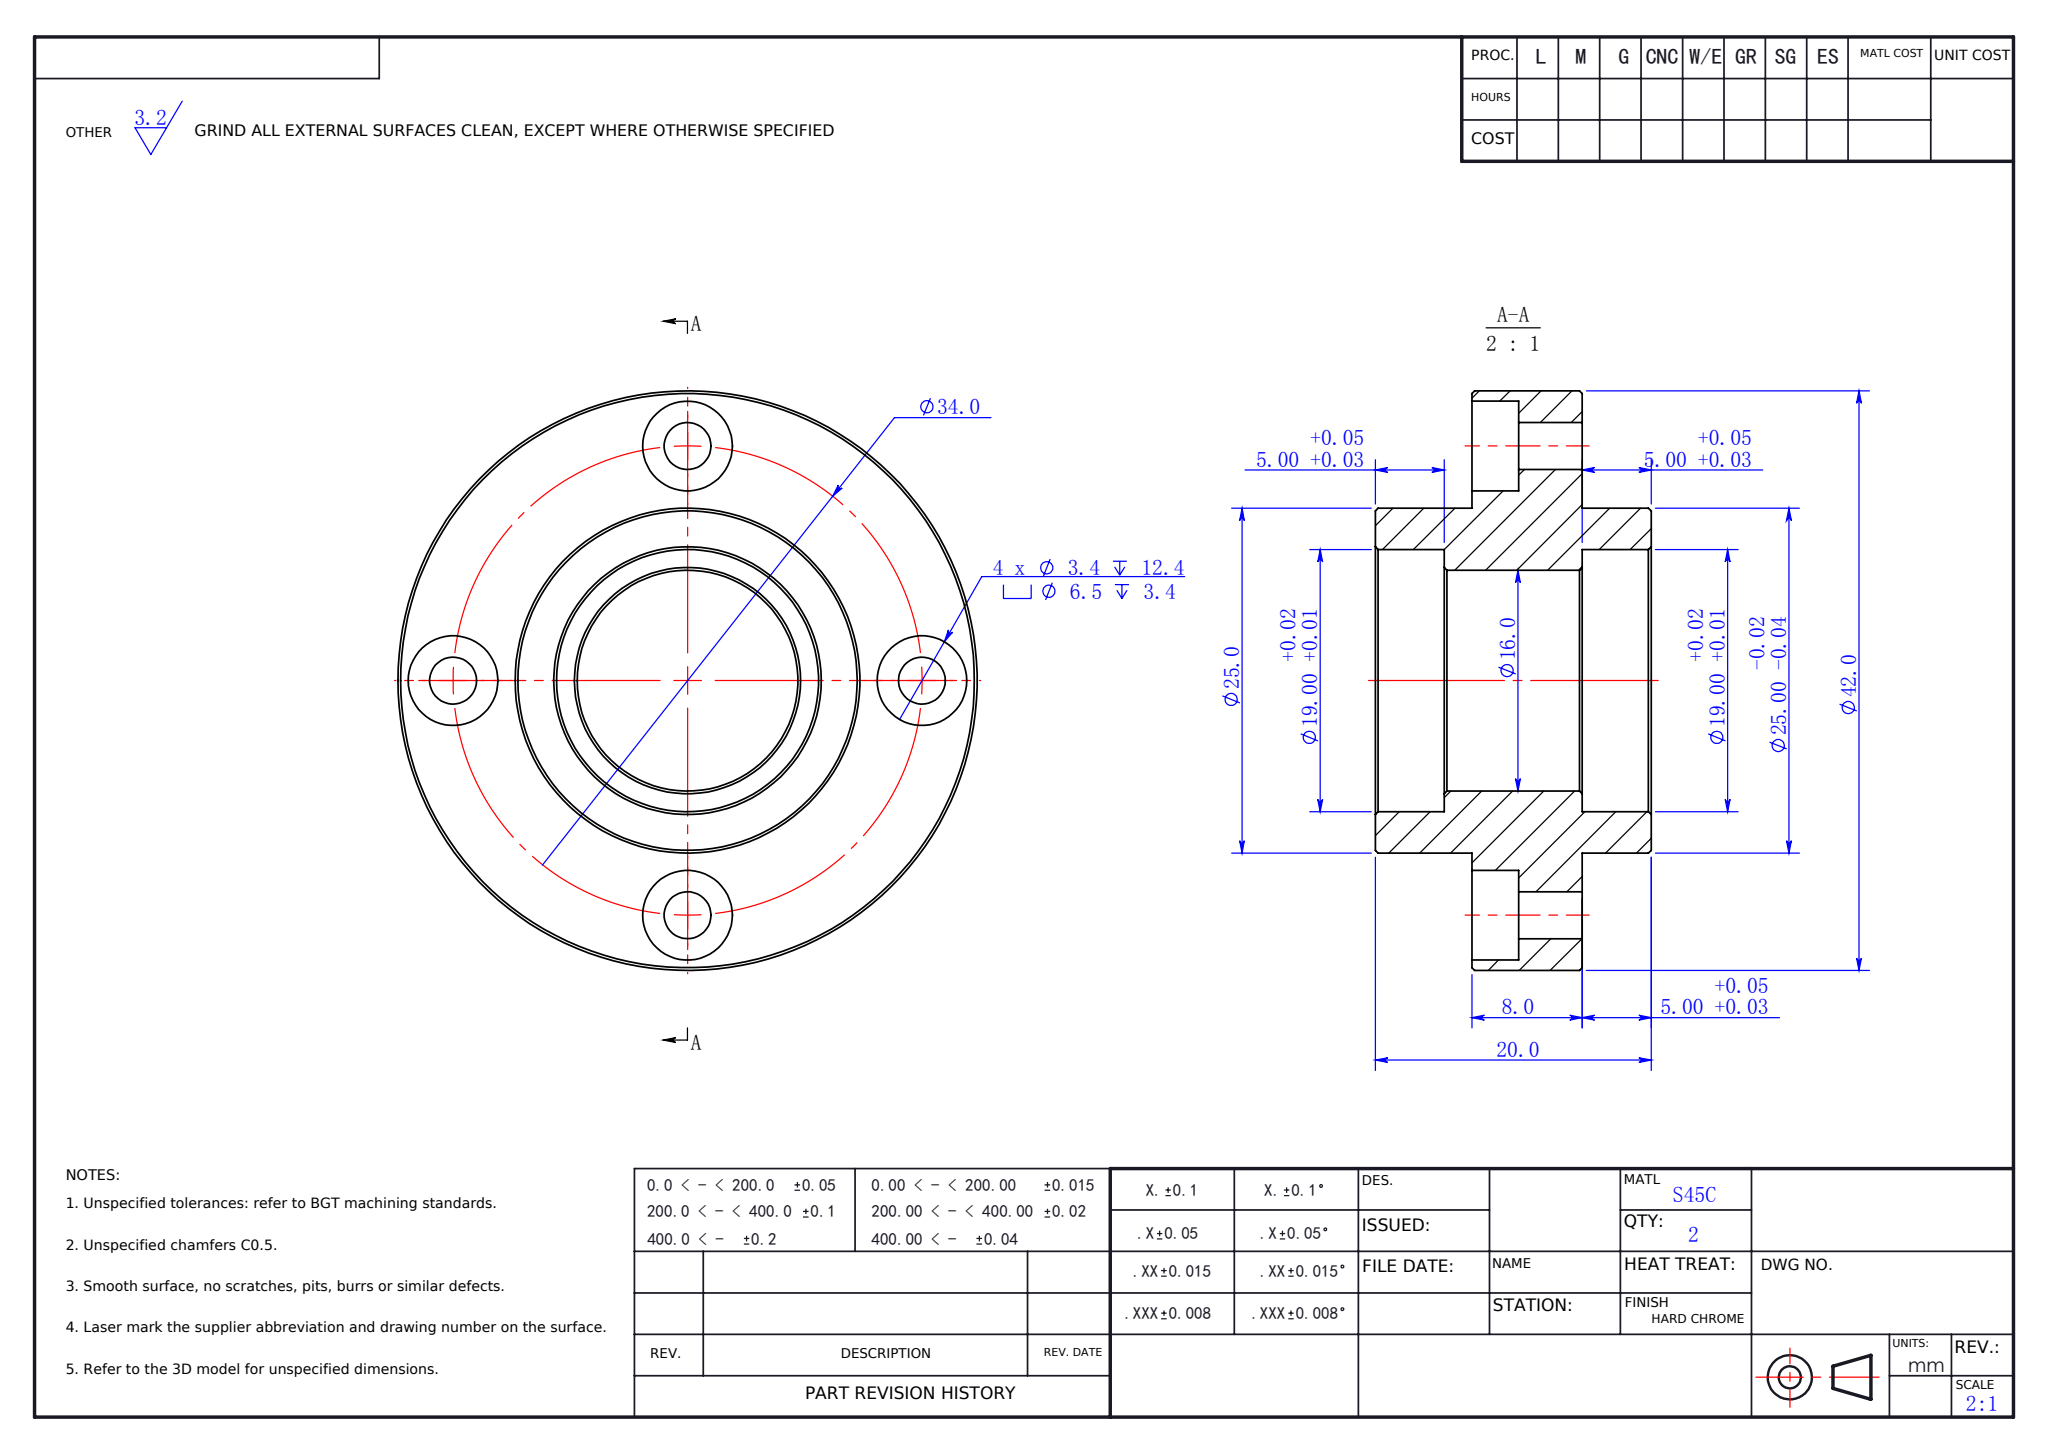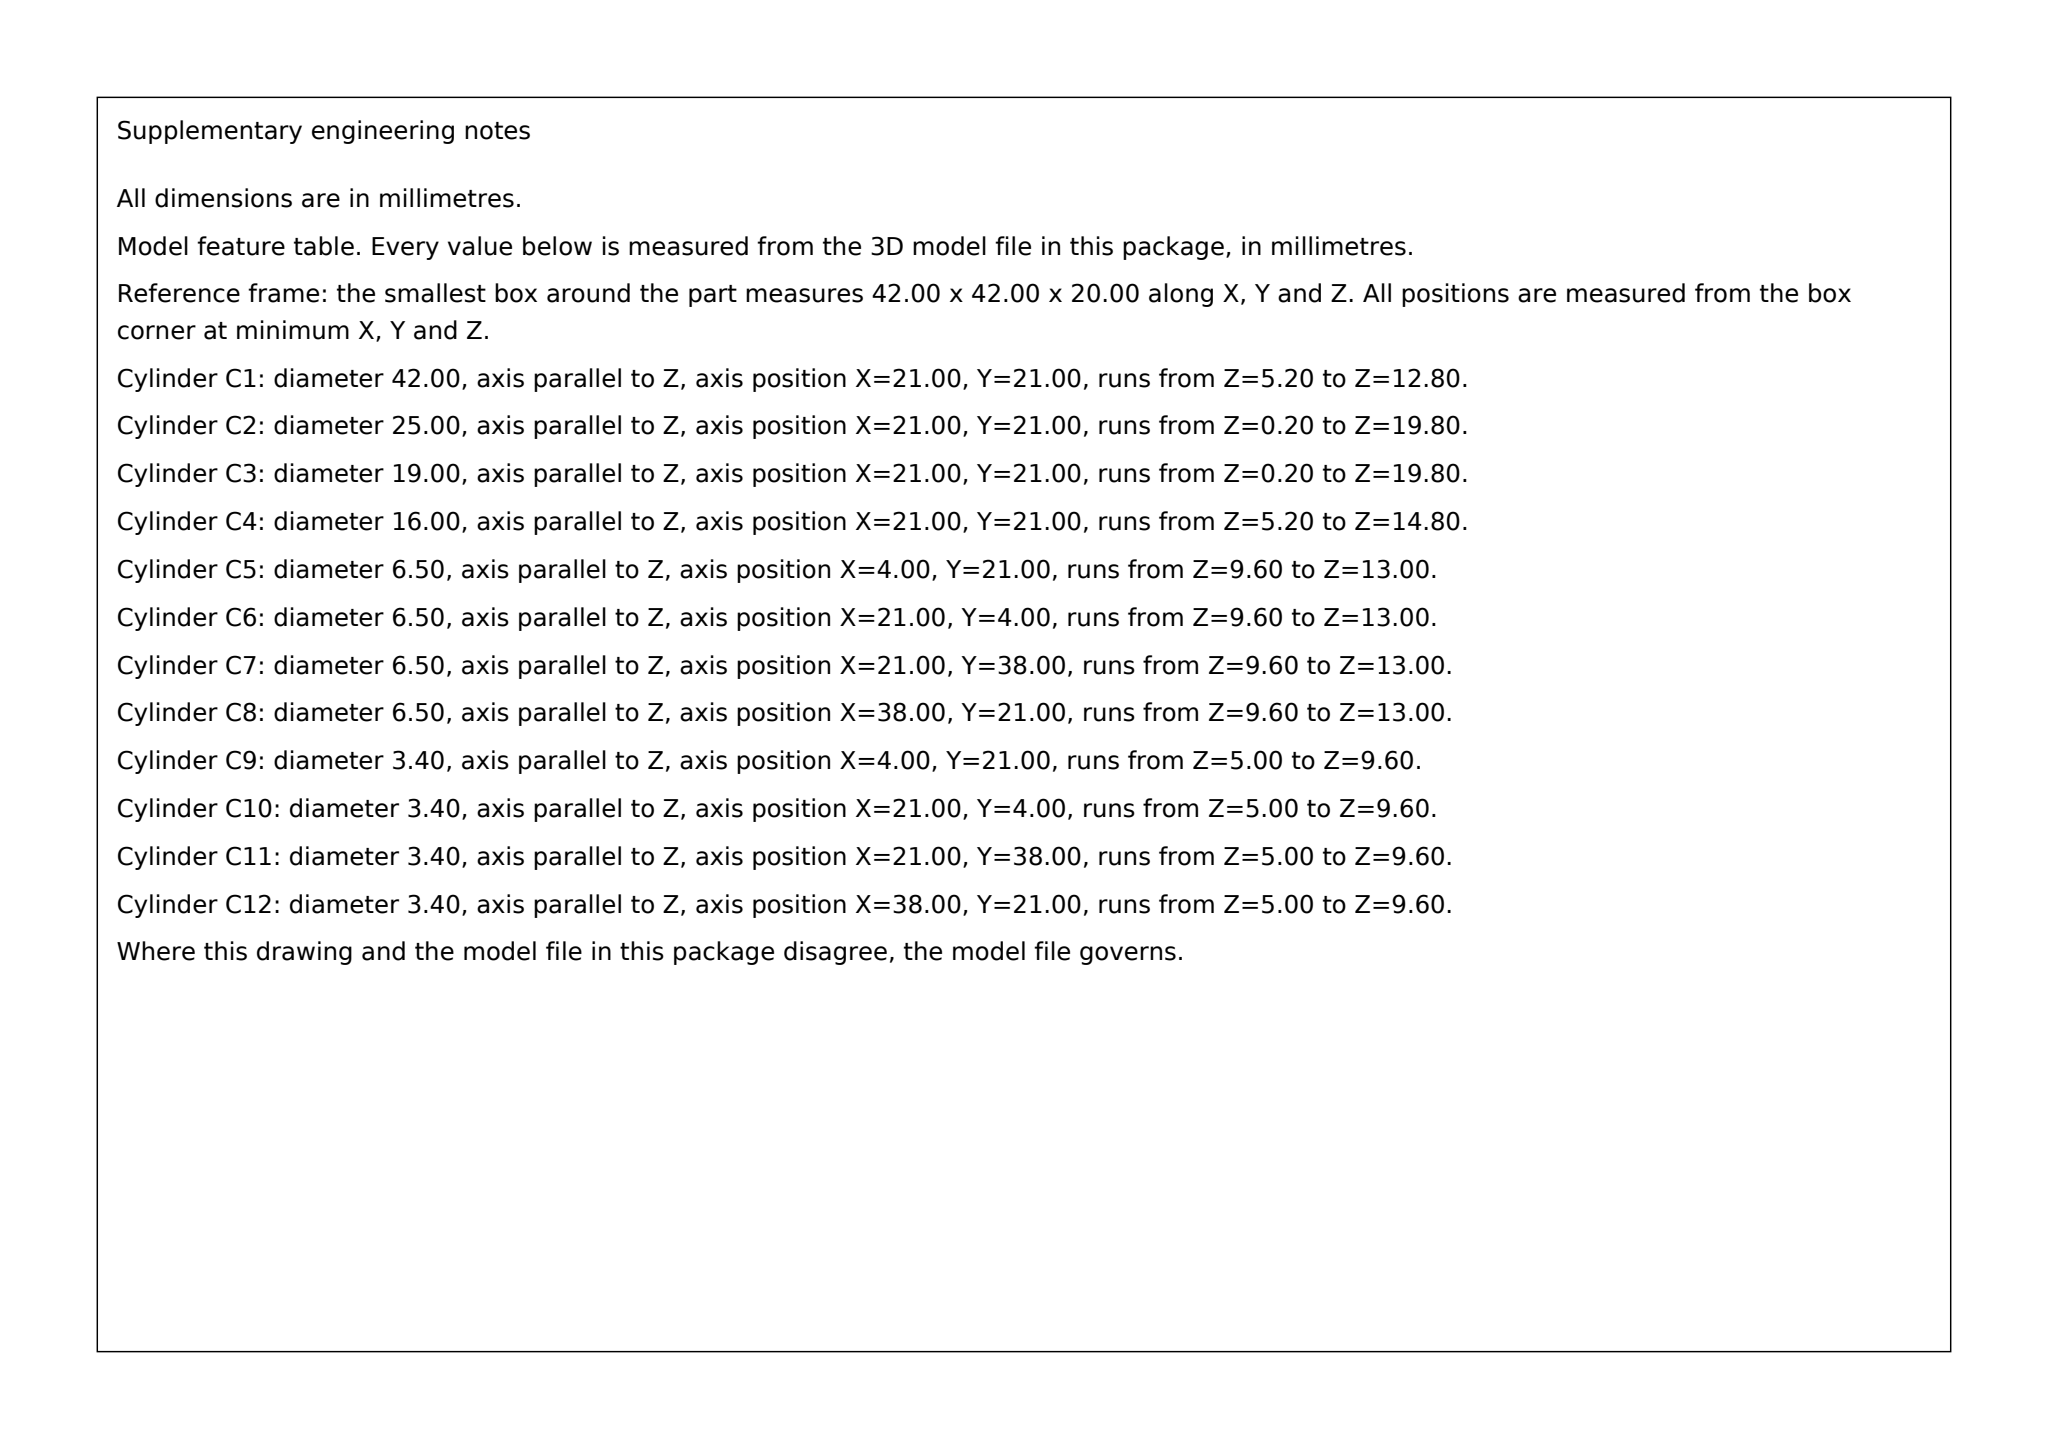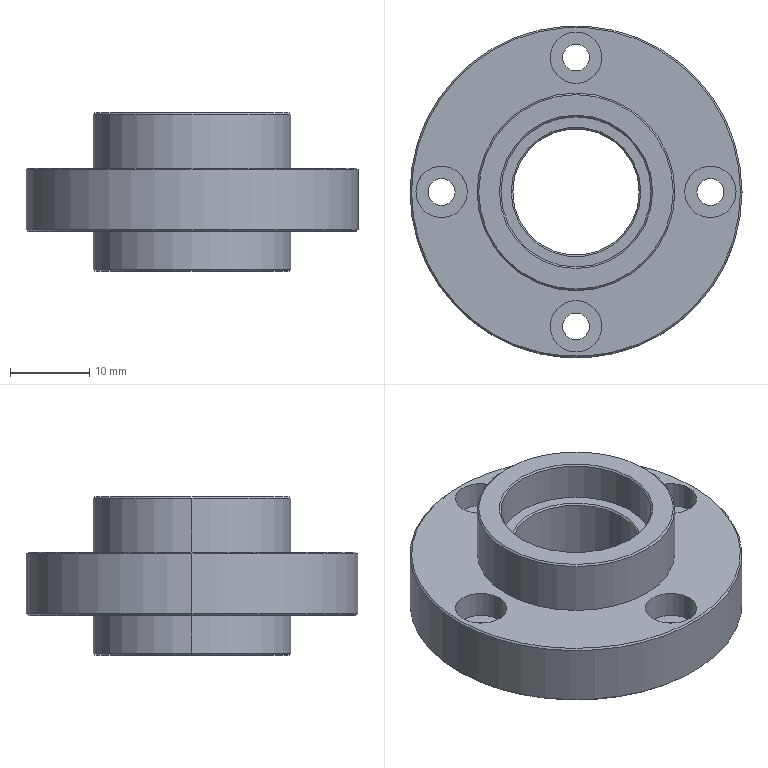Part | SolidWorks | mm | 1 solid | 54 faces | box 42 x 42 x 20 mm | volume 11497 mm3 | cylinder 28 | cone 16 | plane 10 | commonest cylinder face diameters 6.5 x8 3.4 x8 25 x4 19 x4 42 x2 16 x2
build123d program:
from build123d import *

# Parameters (mm, degrees)
CIRPATTERN1_COUNT = 4
CHAMFER1_SIZE     = 0.2


with BuildPart() as part:
    # Sketch1 → Revolve1 (revolve)
    with BuildSketch(Plane(origin=(0, 0, 0), x_dir=(0, 0, -1), z_dir=(1, 0, 0)), mode=Mode.PRIVATE) as revolve1_sk:
        Polygon((0, 9.5), (0, 12.5), (7, 12.5), (7, 21), (15, 21), (15, 12.5), (20, 12.5), (20, 9.5), (15, 9.5), (15, 8), (5, 8), (5, 9.5), align=None)
    revolve(revolve1_sk.sketch.rotate(Axis((0, 0, 0), (0, 0, -1)), 90), axis=Axis((0, 0, 0), (0, 0, -1)))

    # Sketch6 → M3 Hex Socket Head Cap Screw CBORE1 (revolve, cut)
    with BuildSketch(Plane(origin=(0, 17, -7), x_dir=(0, -1, 0), z_dir=(1, 0, 0))):
        Polygon((0, 0), (0, 13.421), (1.7, 12.4), (1.7, 3.4), (3.25, 3.4), (3.25, 0), align=None)
    m3_hex_socket_head_cap_screw_cbore1 = revolve(axis=Axis((0, 17, -0.65), (0, 0, -1)), mode=Mode.SUBTRACT)

    # CirPattern1: M3 Hex Socket Head Cap Screw CBORE1 ×4 about axis
    cirpattern1_axis = Axis((0, 0, 0), (0, 0, 1))
    for i in range(1, CIRPATTERN1_COUNT):
        add(m3_hex_socket_head_cap_screw_cbore1.rotate(cirpattern1_axis, i * 360 / CIRPATTERN1_COUNT), mode=Mode.SUBTRACT)

    # Chamfer1
    chamfer1_edges = [part.edges().sort_by_distance(p)[0] for p in [
        (-12.5, 0, -20),
        (-9.5, 0, -20),
        (-8, 0, -15),
        (-8, 0, -5),
        (-9.5, 0, 0),
        (-12.5, 0, 0),
        (-21, 0, -7),
        (-21, 0, -15),
    ]]
    chamfer(chamfer1_edges, length=CHAMFER1_SIZE)


solid = part.part